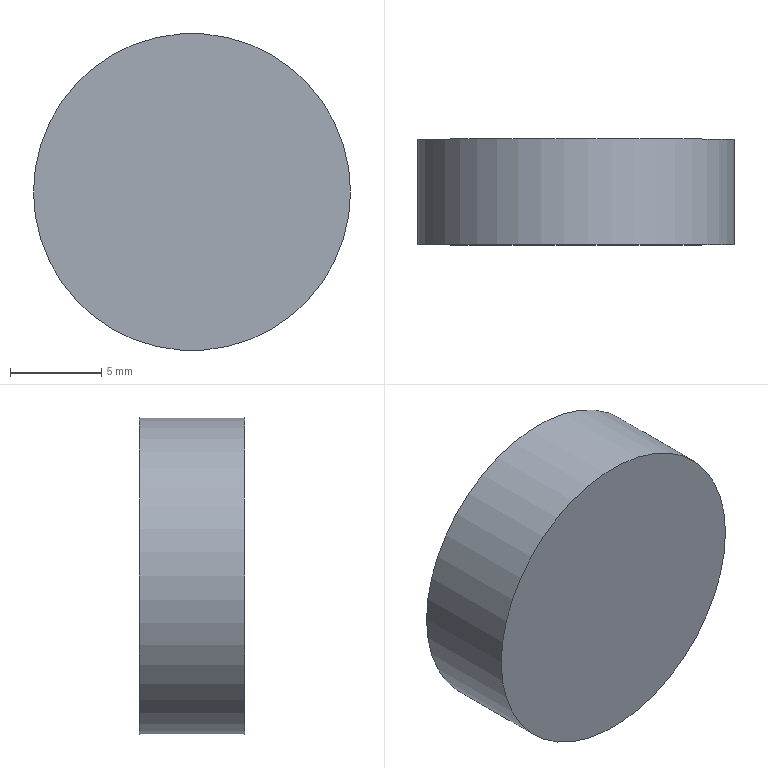Component | NX | VALVE_BODY_FILTER | 1 solid | 3 faces | box 17.4 x 5.8 x 17.4 mm | volume 1379 mm3 | plane 2 | cylinder 1 | commonest cylinder face diameters 17.4 x1
STEP:
#1=CARTESIAN_POINT('',(0.,0.,0.));
#2=DIRECTION('',(0.,0.,1.));
#3=DIRECTION('',(1.,0.,0.));
#4=AXIS2_PLACEMENT_3D('',#1,#2,#3);
#5=CARTESIAN_POINT('',(51.895,48.009,-0.));
#6=VERTEX_POINT('',#5);
#7=CARTESIAN_POINT('',(43.195,48.009,-0.));
#8=DIRECTION('',(0.,-1.,0.));
#9=DIRECTION('',(1.,0.,0.));
#10=AXIS2_PLACEMENT_3D('',#7,#8,#9);
#11=CIRCLE('',#10,8.7);
#12=CARTESIAN_POINT('',(43.195,48.009,-0.));
#13=DIRECTION('',(0.,1.,0.));
#14=DIRECTION('',(-1.,0.,0.));
#15=AXIS2_PLACEMENT_3D('',#12,#13,#14);
#16=CYLINDRICAL_SURFACE('',#15,8.7);
#17=CARTESIAN_POINT('',(9.425,0.));
#18=DIRECTION('',(-1.,0.));
#19=VECTOR('',#18,1.);
#20=LINE('',#17,#19);
#21=(GEOMETRIC_REPRESENTATION_CONTEXT(2)PARAMETRIC_REPRESENTATION_CONTEXT()REPRESENTATION_CONTEXT('',''));
#22=DEFINITIONAL_REPRESENTATION('',(#20),#21);
#23=PCURVE('',#16,#22);
#24=CARTESIAN_POINT('',(43.195,48.009,-0.));
#25=DIRECTION('',(0.,-1.,0.));
#26=DIRECTION('',(1.,0.,0.));
#27=AXIS2_PLACEMENT_3D('',#24,#25,#26);
#28=PLANE('',#27);
#29=CARTESIAN_POINT('',(0.,0.));
#30=DIRECTION('',(1.,0.));
#31=AXIS2_PLACEMENT_2D('',#29,#30);
#32=CIRCLE('',#31,8.7);
#33=(GEOMETRIC_REPRESENTATION_CONTEXT(2)PARAMETRIC_REPRESENTATION_CONTEXT()REPRESENTATION_CONTEXT('',''));
#34=DEFINITIONAL_REPRESENTATION('',(#32),#33);
#35=PCURVE('',#28,#34);
#36=SURFACE_CURVE('',#11,(#23,#35),.PCURVE_S1.);
#37=EDGE_CURVE('',#6,#6,#36,.T.);
#38=ORIENTED_EDGE('',*,*,#37,.F.);
#39=CARTESIAN_POINT('',(51.895,53.809,-0.));
#40=VERTEX_POINT('',#39);
#41=CARTESIAN_POINT('',(51.895,48.009,0.));
#42=CARTESIAN_POINT('',(51.895,53.809,0.));
#43=B_SPLINE_CURVE_WITH_KNOTS('',1,(#41,#42),.UNSPECIFIED.,.F.,.F.,(2,2),(0.,5.8),.PIECEWISE_BEZIER_KNOTS.);
#44=CARTESIAN_POINT('',(9.425,0.));
#45=DIRECTION('',(0.,1.));
#46=VECTOR('',#45,1.);
#47=LINE('',#44,#46);
#48=(GEOMETRIC_REPRESENTATION_CONTEXT(2)PARAMETRIC_REPRESENTATION_CONTEXT()REPRESENTATION_CONTEXT('',''));
#49=DEFINITIONAL_REPRESENTATION('',(#47),#48);
#50=PCURVE('',#16,#49);
#51=CARTESIAN_POINT('',(3.142,0.));
#52=DIRECTION('',(0.,1.));
#53=VECTOR('',#52,1.);
#54=LINE('',#51,#53);
#55=(GEOMETRIC_REPRESENTATION_CONTEXT(2)PARAMETRIC_REPRESENTATION_CONTEXT()REPRESENTATION_CONTEXT('',''));
#56=DEFINITIONAL_REPRESENTATION('',(#54),#55);
#57=PCURVE('',#16,#56);
#58=SEAM_CURVE('',#43,(#50,#57),.PCURVE_S1.);
#59=EDGE_CURVE('',#6,#40,#58,.T.);
#60=ORIENTED_EDGE('',*,*,#59,.T.);
#61=CARTESIAN_POINT('',(43.195,53.809,-0.));
#62=DIRECTION('',(0.,-1.,0.));
#63=DIRECTION('',(1.,0.,0.));
#64=AXIS2_PLACEMENT_3D('',#61,#62,#63);
#65=CIRCLE('',#64,8.7);
#66=CARTESIAN_POINT('',(9.425,5.8));
#67=DIRECTION('',(-1.,0.));
#68=VECTOR('',#67,1.);
#69=LINE('',#66,#68);
#70=(GEOMETRIC_REPRESENTATION_CONTEXT(2)PARAMETRIC_REPRESENTATION_CONTEXT()REPRESENTATION_CONTEXT('',''));
#71=DEFINITIONAL_REPRESENTATION('',(#69),#70);
#72=PCURVE('',#16,#71);
#73=CARTESIAN_POINT('',(43.195,53.809,-0.));
#74=DIRECTION('',(0.,-1.,0.));
#75=DIRECTION('',(1.,0.,0.));
#76=AXIS2_PLACEMENT_3D('',#73,#74,#75);
#77=PLANE('',#76);
#78=CARTESIAN_POINT('',(0.,0.));
#79=DIRECTION('',(1.,0.));
#80=AXIS2_PLACEMENT_2D('',#78,#79);
#81=CIRCLE('',#80,8.7);
#82=(GEOMETRIC_REPRESENTATION_CONTEXT(2)PARAMETRIC_REPRESENTATION_CONTEXT()REPRESENTATION_CONTEXT('',''));
#83=DEFINITIONAL_REPRESENTATION('',(#81),#82);
#84=PCURVE('',#77,#83);
#85=SURFACE_CURVE('',#65,(#72,#84),.PCURVE_S1.);
#86=EDGE_CURVE('',#40,#40,#85,.T.);
#87=ORIENTED_EDGE('',*,*,#86,.T.);
#88=ORIENTED_EDGE('',*,*,#59,.F.);
#89=EDGE_LOOP('',(#38,#60,#87,#88));
#90=FACE_BOUND('',#89,.T.);
#91=ADVANCED_FACE('',(#90),#16,.T.);
#92=ORIENTED_EDGE('',*,*,#37,.T.);
#93=EDGE_LOOP('',(#92));
#94=FACE_BOUND('',#93,.T.);
#95=ADVANCED_FACE('',(#94),#28,.T.);
#96=ORIENTED_EDGE('',*,*,#86,.F.);
#97=EDGE_LOOP('',(#96));
#98=FACE_BOUND('',#97,.T.);
#99=ADVANCED_FACE('',(#98),#77,.F.);
#100=CLOSED_SHELL('',(#91,#95,#99));
#101=MANIFOLD_SOLID_BREP('',#100);
#102=(LENGTH_UNIT()NAMED_UNIT(*)SI_UNIT(.MILLI.,.METRE.));
#103=UNCERTAINTY_MEASURE_WITH_UNIT(LENGTH_MEASURE(0.00001),#102,'','');
#104=(NAMED_UNIT(*)PLANE_ANGLE_UNIT()SI_UNIT($,.RADIAN.));
#105=(NAMED_UNIT(*)SI_UNIT($,.STERADIAN.)SOLID_ANGLE_UNIT());
#106=(GEOMETRIC_REPRESENTATION_CONTEXT(3)GLOBAL_UNCERTAINTY_ASSIGNED_CONTEXT((#103))GLOBAL_UNIT_ASSIGNED_CONTEXT((#102,#104,#105))REPRESENTATION_CONTEXT('',''));
#107=ADVANCED_BREP_SHAPE_REPRESENTATION('',(#4,#101),#106);